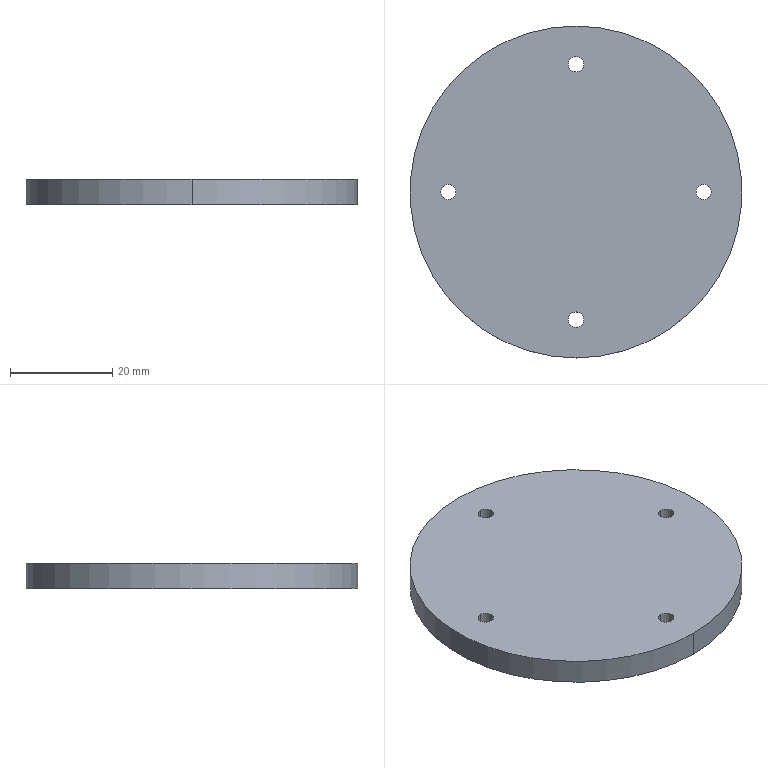Component | SolidWorks | Gimbal-1_GimbalMiddle-1 | 1 solid | 12 faces | box 65 x 65 x 5 mm | volume 16450 mm3 | cylinder 10 | plane 2 | commonest cylinder face diameters 3 x8 65 x2
build123d program:
from build123d import *

# Parameters (mm, degrees)
SKETCH1_R           = 32.5
BOSS_EXTRUDE1_DEPTH = 5
SKETCH2_R           = 1.5
CUT_EXTRUDE3_DEPTH  = 10


with BuildPart() as part:
    # Sketch1 → Boss-Extrude1 (new body)
    with BuildSketch(Plane.XY):
        Circle(SKETCH1_R)
    extrude(amount=BOSS_EXTRUDE1_DEPTH)

    # Sketch2 → Cut-Extrude3 (cut)
    with BuildSketch(Plane.XY.offset(5)):
        with Locations((0, 25)):
            Circle(SKETCH2_R)
        with Locations((25, 0)):
            Circle(SKETCH2_R)
        with Locations((0, -25)):
            Circle(SKETCH2_R)
        with Locations((-25, 0)):
            Circle(SKETCH2_R)
    extrude(amount=-CUT_EXTRUDE3_DEPTH, mode=Mode.SUBTRACT)


solid = part.part

# Placed as in the assembly
solid = solid.moved(Location((0, 96.5, -37), (0, 0, 0)))
STEP:
#1=COLOUR_RGB('',0.7922,0.8196,0.9333);
#2=FILL_AREA_STYLE_COLOUR('',#1);
#3=FILL_AREA_STYLE('',(#2));
#4=SURFACE_STYLE_FILL_AREA(#3);
#5=SURFACE_SIDE_STYLE('',(#4));
#6=SURFACE_STYLE_USAGE(.BOTH.,#5);
#7=PRESENTATION_STYLE_ASSIGNMENT((#6));
#8=CARTESIAN_POINT('',(-0.9843,3.858,-1.26));
#9=VERTEX_POINT('',#8);
#10=CARTESIAN_POINT('',(-0.9843,3.74,-1.26));
#11=VERTEX_POINT('',#10);
#12=CARTESIAN_POINT('',(-0.9843,3.799,-1.26));
#13=DIRECTION('',(0.,0.,-1.));
#14=DIRECTION('',(0.,-1.,0.));
#15=AXIS2_PLACEMENT_3D('',#12,#13,#14);
#16=CIRCLE('',#15,0.05906);
#17=EDGE_CURVE('',#9,#11,#16,.T.);
#18=ORIENTED_EDGE('',*,*,#17,.F.);
#19=CARTESIAN_POINT('',(-0.9843,3.858,-1.457));
#20=VERTEX_POINT('',#19);
#21=CARTESIAN_POINT('',(-0.9843,3.858,-1.063));
#22=DIRECTION('',(0.,0.,-1.));
#23=VECTOR('',#22,39.37);
#24=LINE('',#21,#23);
#25=EDGE_CURVE('',#9,#20,#24,.T.);
#26=ORIENTED_EDGE('',*,*,#25,.T.);
#27=CARTESIAN_POINT('',(-0.9843,3.74,-1.457));
#28=VERTEX_POINT('',#27);
#29=CARTESIAN_POINT('',(-0.9843,3.799,-1.457));
#30=DIRECTION('',(0.,0.,-1.));
#31=DIRECTION('',(0.,-1.,0.));
#32=AXIS2_PLACEMENT_3D('',#29,#30,#31);
#33=CIRCLE('',#32,0.05906);
#34=EDGE_CURVE('',#20,#28,#33,.T.);
#35=ORIENTED_EDGE('',*,*,#34,.T.);
#36=CARTESIAN_POINT('',(-0.9843,3.74,-1.063));
#37=DIRECTION('',(0.,0.,-1.));
#38=VECTOR('',#37,39.37);
#39=LINE('',#36,#38);
#40=EDGE_CURVE('',#11,#28,#39,.T.);
#41=ORIENTED_EDGE('',*,*,#40,.F.);
#42=EDGE_LOOP('',(#18,#26,#35,#41));
#43=FACE_OUTER_BOUND('',#42,.T.);
#44=CARTESIAN_POINT('',(-0.9843,3.799,-1.063));
#45=DIRECTION('',(0.,0.,-1.));
#46=DIRECTION('',(0.,-1.,0.));
#47=AXIS2_PLACEMENT_3D('',#44,#45,#46);
#48=CYLINDRICAL_SURFACE('',#47,0.05906);
#49=ADVANCED_FACE('',(#43),#48,.F.);
#50=CARTESIAN_POINT('',(0.,2.874,-1.26));
#51=VERTEX_POINT('',#50);
#52=CARTESIAN_POINT('',(0.,2.756,-1.26));
#53=VERTEX_POINT('',#52);
#54=CARTESIAN_POINT('',(0.,2.815,-1.26));
#55=DIRECTION('',(0.,0.,-1.));
#56=DIRECTION('',(0.,-1.,0.));
#57=AXIS2_PLACEMENT_3D('',#54,#55,#56);
#58=CIRCLE('',#57,0.05906);
#59=EDGE_CURVE('',#51,#53,#58,.T.);
#60=ORIENTED_EDGE('',*,*,#59,.F.);
#61=CARTESIAN_POINT('',(0.,2.874,-1.457));
#62=VERTEX_POINT('',#61);
#63=CARTESIAN_POINT('',(0.,2.874,-1.063));
#64=DIRECTION('',(0.,0.,-1.));
#65=VECTOR('',#64,39.37);
#66=LINE('',#63,#65);
#67=EDGE_CURVE('',#51,#62,#66,.T.);
#68=ORIENTED_EDGE('',*,*,#67,.T.);
#69=CARTESIAN_POINT('',(0.,2.756,-1.457));
#70=VERTEX_POINT('',#69);
#71=CARTESIAN_POINT('',(0.,2.815,-1.457));
#72=DIRECTION('',(0.,0.,-1.));
#73=DIRECTION('',(0.,-1.,0.));
#74=AXIS2_PLACEMENT_3D('',#71,#72,#73);
#75=CIRCLE('',#74,0.05906);
#76=EDGE_CURVE('',#62,#70,#75,.T.);
#77=ORIENTED_EDGE('',*,*,#76,.T.);
#78=CARTESIAN_POINT('',(0.,2.756,-1.063));
#79=DIRECTION('',(0.,0.,-1.));
#80=VECTOR('',#79,39.37);
#81=LINE('',#78,#80);
#82=EDGE_CURVE('',#53,#70,#81,.T.);
#83=ORIENTED_EDGE('',*,*,#82,.F.);
#84=EDGE_LOOP('',(#60,#68,#77,#83));
#85=FACE_OUTER_BOUND('',#84,.T.);
#86=CARTESIAN_POINT('',(0.,2.815,-1.063));
#87=DIRECTION('',(0.,0.,-1.));
#88=DIRECTION('',(0.,-1.,0.));
#89=AXIS2_PLACEMENT_3D('',#86,#87,#88);
#90=CYLINDRICAL_SURFACE('',#89,0.05906);
#91=ADVANCED_FACE('',(#85),#90,.F.);
#92=CARTESIAN_POINT('',(0.9843,3.858,-1.26));
#93=VERTEX_POINT('',#92);
#94=CARTESIAN_POINT('',(0.9843,3.74,-1.26));
#95=VERTEX_POINT('',#94);
#96=CARTESIAN_POINT('',(0.9843,3.799,-1.26));
#97=DIRECTION('',(0.,0.,-1.));
#98=DIRECTION('',(0.,-1.,0.));
#99=AXIS2_PLACEMENT_3D('',#96,#97,#98);
#100=CIRCLE('',#99,0.05906);
#101=EDGE_CURVE('',#93,#95,#100,.T.);
#102=ORIENTED_EDGE('',*,*,#101,.F.);
#103=CARTESIAN_POINT('',(0.9843,3.858,-1.457));
#104=VERTEX_POINT('',#103);
#105=CARTESIAN_POINT('',(0.9843,3.858,-1.063));
#106=DIRECTION('',(0.,0.,-1.));
#107=VECTOR('',#106,39.37);
#108=LINE('',#105,#107);
#109=EDGE_CURVE('',#93,#104,#108,.T.);
#110=ORIENTED_EDGE('',*,*,#109,.T.);
#111=CARTESIAN_POINT('',(0.9843,3.74,-1.457));
#112=VERTEX_POINT('',#111);
#113=CARTESIAN_POINT('',(0.9843,3.799,-1.457));
#114=DIRECTION('',(0.,0.,-1.));
#115=DIRECTION('',(0.,-1.,0.));
#116=AXIS2_PLACEMENT_3D('',#113,#114,#115);
#117=CIRCLE('',#116,0.05906);
#118=EDGE_CURVE('',#104,#112,#117,.T.);
#119=ORIENTED_EDGE('',*,*,#118,.T.);
#120=CARTESIAN_POINT('',(0.9843,3.74,-1.063));
#121=DIRECTION('',(0.,0.,-1.));
#122=VECTOR('',#121,39.37);
#123=LINE('',#120,#122);
#124=EDGE_CURVE('',#95,#112,#123,.T.);
#125=ORIENTED_EDGE('',*,*,#124,.F.);
#126=EDGE_LOOP('',(#102,#110,#119,#125));
#127=FACE_OUTER_BOUND('',#126,.T.);
#128=CARTESIAN_POINT('',(0.9843,3.799,-1.063));
#129=DIRECTION('',(0.,0.,-1.));
#130=DIRECTION('',(0.,-1.,0.));
#131=AXIS2_PLACEMENT_3D('',#128,#129,#130);
#132=CYLINDRICAL_SURFACE('',#131,0.05906);
#133=ADVANCED_FACE('',(#127),#132,.F.);
#134=CARTESIAN_POINT('',(-0.,4.843,-1.26));
#135=VERTEX_POINT('',#134);
#136=CARTESIAN_POINT('',(-0.,4.724,-1.26));
#137=VERTEX_POINT('',#136);
#138=CARTESIAN_POINT('',(-0.,4.783,-1.26));
#139=DIRECTION('',(0.,0.,-1.));
#140=DIRECTION('',(0.,-1.,0.));
#141=AXIS2_PLACEMENT_3D('',#138,#139,#140);
#142=CIRCLE('',#141,0.05906);
#143=EDGE_CURVE('',#135,#137,#142,.T.);
#144=ORIENTED_EDGE('',*,*,#143,.F.);
#145=CARTESIAN_POINT('',(-0.,4.843,-1.457));
#146=VERTEX_POINT('',#145);
#147=CARTESIAN_POINT('',(-0.,4.843,-1.063));
#148=DIRECTION('',(0.,0.,-1.));
#149=VECTOR('',#148,39.37);
#150=LINE('',#147,#149);
#151=EDGE_CURVE('',#135,#146,#150,.T.);
#152=ORIENTED_EDGE('',*,*,#151,.T.);
#153=CARTESIAN_POINT('',(-0.,4.724,-1.457));
#154=VERTEX_POINT('',#153);
#155=CARTESIAN_POINT('',(-0.,4.783,-1.457));
#156=DIRECTION('',(0.,0.,-1.));
#157=DIRECTION('',(0.,-1.,0.));
#158=AXIS2_PLACEMENT_3D('',#155,#156,#157);
#159=CIRCLE('',#158,0.05906);
#160=EDGE_CURVE('',#146,#154,#159,.T.);
#161=ORIENTED_EDGE('',*,*,#160,.T.);
#162=CARTESIAN_POINT('',(-0.,4.724,-1.063));
#163=DIRECTION('',(0.,0.,-1.));
#164=VECTOR('',#163,39.37);
#165=LINE('',#162,#164);
#166=EDGE_CURVE('',#137,#154,#165,.T.);
#167=ORIENTED_EDGE('',*,*,#166,.F.);
#168=EDGE_LOOP('',(#144,#152,#161,#167));
#169=FACE_OUTER_BOUND('',#168,.T.);
#170=CARTESIAN_POINT('',(-0.,4.783,-1.063));
#171=DIRECTION('',(0.,0.,-1.));
#172=DIRECTION('',(0.,-1.,0.));
#173=AXIS2_PLACEMENT_3D('',#170,#171,#172);
#174=CYLINDRICAL_SURFACE('',#173,0.05906);
#175=ADVANCED_FACE('',(#169),#174,.F.);
#176=CARTESIAN_POINT('',(0.,2.52,-1.457));
#177=VERTEX_POINT('',#176);
#178=CARTESIAN_POINT('',(-0.,5.079,-1.457));
#179=VERTEX_POINT('',#178);
#180=CARTESIAN_POINT('',(0.,3.799,-1.457));
#181=DIRECTION('',(0.,0.,-1.));
#182=DIRECTION('',(0.,-1.,0.));
#183=AXIS2_PLACEMENT_3D('',#180,#181,#182);
#184=CIRCLE('',#183,1.28);
#185=EDGE_CURVE('',#177,#179,#184,.T.);
#186=ORIENTED_EDGE('',*,*,#185,.F.);
#187=CARTESIAN_POINT('',(0.,2.52,-1.26));
#188=VERTEX_POINT('',#187);
#189=CARTESIAN_POINT('',(0.,2.52,-1.457));
#190=DIRECTION('',(0.,0.,1.));
#191=VECTOR('',#190,39.37);
#192=LINE('',#189,#191);
#193=EDGE_CURVE('',#177,#188,#192,.T.);
#194=ORIENTED_EDGE('',*,*,#193,.T.);
#195=CARTESIAN_POINT('',(-0.,5.079,-1.26));
#196=VERTEX_POINT('',#195);
#197=CARTESIAN_POINT('',(0.,3.799,-1.26));
#198=DIRECTION('',(0.,0.,-1.));
#199=DIRECTION('',(0.,-1.,0.));
#200=AXIS2_PLACEMENT_3D('',#197,#198,#199);
#201=CIRCLE('',#200,1.28);
#202=EDGE_CURVE('',#188,#196,#201,.T.);
#203=ORIENTED_EDGE('',*,*,#202,.T.);
#204=CARTESIAN_POINT('',(-0.,5.079,-1.457));
#205=DIRECTION('',(0.,0.,1.));
#206=VECTOR('',#205,39.37);
#207=LINE('',#204,#206);
#208=EDGE_CURVE('',#179,#196,#207,.T.);
#209=ORIENTED_EDGE('',*,*,#208,.F.);
#210=EDGE_LOOP('',(#186,#194,#203,#209));
#211=FACE_OUTER_BOUND('',#210,.T.);
#212=CARTESIAN_POINT('',(0.,3.799,-1.457));
#213=DIRECTION('',(0.,0.,1.));
#214=DIRECTION('',(-0.,1.,0.));
#215=AXIS2_PLACEMENT_3D('',#212,#213,#214);
#216=CYLINDRICAL_SURFACE('',#215,1.28);
#217=ADVANCED_FACE('',(#211),#216,.T.);
#218=ORIENTED_EDGE('',*,*,#193,.F.);
#219=CARTESIAN_POINT('',(0.,3.799,-1.457));
#220=DIRECTION('',(0.,0.,-1.));
#221=DIRECTION('',(0.,-1.,0.));
#222=AXIS2_PLACEMENT_3D('',#219,#220,#221);
#223=CIRCLE('',#222,1.28);
#224=EDGE_CURVE('',#179,#177,#223,.T.);
#225=ORIENTED_EDGE('',*,*,#224,.F.);
#226=ORIENTED_EDGE('',*,*,#208,.T.);
#227=CARTESIAN_POINT('',(0.,3.799,-1.26));
#228=DIRECTION('',(0.,0.,-1.));
#229=DIRECTION('',(0.,-1.,0.));
#230=AXIS2_PLACEMENT_3D('',#227,#228,#229);
#231=CIRCLE('',#230,1.28);
#232=EDGE_CURVE('',#196,#188,#231,.T.);
#233=ORIENTED_EDGE('',*,*,#232,.T.);
#234=EDGE_LOOP('',(#218,#225,#226,#233));
#235=FACE_OUTER_BOUND('',#234,.T.);
#236=CARTESIAN_POINT('',(0.,3.799,-1.457));
#237=DIRECTION('',(0.,0.,1.));
#238=DIRECTION('',(-0.,1.,0.));
#239=AXIS2_PLACEMENT_3D('',#236,#237,#238);
#240=CYLINDRICAL_SURFACE('',#239,1.28);
#241=ADVANCED_FACE('',(#235),#240,.T.);
#242=CARTESIAN_POINT('',(-0.9843,3.799,-1.457));
#243=DIRECTION('',(0.,0.,-1.));
#244=DIRECTION('',(0.,-1.,0.));
#245=AXIS2_PLACEMENT_3D('',#242,#243,#244);
#246=CIRCLE('',#245,0.05906);
#247=EDGE_CURVE('',#28,#20,#246,.T.);
#248=ORIENTED_EDGE('',*,*,#247,.F.);
#249=ORIENTED_EDGE('',*,*,#34,.F.);
#250=EDGE_LOOP('',(#248,#249));
#251=FACE_BOUND('',#250,.T.);
#252=CARTESIAN_POINT('',(0.,2.815,-1.457));
#253=DIRECTION('',(0.,0.,-1.));
#254=DIRECTION('',(0.,-1.,0.));
#255=AXIS2_PLACEMENT_3D('',#252,#253,#254);
#256=CIRCLE('',#255,0.05906);
#257=EDGE_CURVE('',#70,#62,#256,.T.);
#258=ORIENTED_EDGE('',*,*,#257,.F.);
#259=ORIENTED_EDGE('',*,*,#76,.F.);
#260=EDGE_LOOP('',(#258,#259));
#261=FACE_BOUND('',#260,.T.);
#262=CARTESIAN_POINT('',(0.9843,3.799,-1.457));
#263=DIRECTION('',(0.,0.,-1.));
#264=DIRECTION('',(0.,-1.,0.));
#265=AXIS2_PLACEMENT_3D('',#262,#263,#264);
#266=CIRCLE('',#265,0.05906);
#267=EDGE_CURVE('',#112,#104,#266,.T.);
#268=ORIENTED_EDGE('',*,*,#267,.F.);
#269=ORIENTED_EDGE('',*,*,#118,.F.);
#270=EDGE_LOOP('',(#268,#269));
#271=FACE_BOUND('',#270,.T.);
#272=CARTESIAN_POINT('',(-0.,4.783,-1.457));
#273=DIRECTION('',(0.,0.,-1.));
#274=DIRECTION('',(0.,-1.,0.));
#275=AXIS2_PLACEMENT_3D('',#272,#273,#274);
#276=CIRCLE('',#275,0.05906);
#277=EDGE_CURVE('',#154,#146,#276,.T.);
#278=ORIENTED_EDGE('',*,*,#277,.F.);
#279=ORIENTED_EDGE('',*,*,#160,.F.);
#280=EDGE_LOOP('',(#278,#279));
#281=FACE_BOUND('',#280,.T.);
#282=ORIENTED_EDGE('',*,*,#224,.T.);
#283=ORIENTED_EDGE('',*,*,#185,.T.);
#284=EDGE_LOOP('',(#282,#283));
#285=FACE_OUTER_BOUND('',#284,.T.);
#286=CARTESIAN_POINT('',(0.,3.799,-1.457));
#287=DIRECTION('',(0.,0.,-1.));
#288=DIRECTION('',(0.,-1.,0.));
#289=AXIS2_PLACEMENT_3D('',#286,#287,#288);
#290=PLANE('',#289);
#291=ADVANCED_FACE('',(#251,#261,#271,#281,#285),#290,.T.);
#292=CARTESIAN_POINT('',(-0.9843,3.799,-1.26));
#293=DIRECTION('',(0.,0.,-1.));
#294=DIRECTION('',(0.,-1.,0.));
#295=AXIS2_PLACEMENT_3D('',#292,#293,#294);
#296=CIRCLE('',#295,0.05906);
#297=EDGE_CURVE('',#11,#9,#296,.T.);
#298=ORIENTED_EDGE('',*,*,#297,.T.);
#299=ORIENTED_EDGE('',*,*,#17,.T.);
#300=EDGE_LOOP('',(#298,#299));
#301=FACE_BOUND('',#300,.T.);
#302=CARTESIAN_POINT('',(0.,2.815,-1.26));
#303=DIRECTION('',(0.,0.,-1.));
#304=DIRECTION('',(0.,-1.,0.));
#305=AXIS2_PLACEMENT_3D('',#302,#303,#304);
#306=CIRCLE('',#305,0.05906);
#307=EDGE_CURVE('',#53,#51,#306,.T.);
#308=ORIENTED_EDGE('',*,*,#307,.T.);
#309=ORIENTED_EDGE('',*,*,#59,.T.);
#310=EDGE_LOOP('',(#308,#309));
#311=FACE_BOUND('',#310,.T.);
#312=CARTESIAN_POINT('',(0.9843,3.799,-1.26));
#313=DIRECTION('',(0.,0.,-1.));
#314=DIRECTION('',(0.,-1.,0.));
#315=AXIS2_PLACEMENT_3D('',#312,#313,#314);
#316=CIRCLE('',#315,0.05906);
#317=EDGE_CURVE('',#95,#93,#316,.T.);
#318=ORIENTED_EDGE('',*,*,#317,.T.);
#319=ORIENTED_EDGE('',*,*,#101,.T.);
#320=EDGE_LOOP('',(#318,#319));
#321=FACE_BOUND('',#320,.T.);
#322=CARTESIAN_POINT('',(-0.,4.783,-1.26));
#323=DIRECTION('',(0.,0.,-1.));
#324=DIRECTION('',(0.,-1.,0.));
#325=AXIS2_PLACEMENT_3D('',#322,#323,#324);
#326=CIRCLE('',#325,0.05906);
#327=EDGE_CURVE('',#137,#135,#326,.T.);
#328=ORIENTED_EDGE('',*,*,#327,.T.);
#329=ORIENTED_EDGE('',*,*,#143,.T.);
#330=EDGE_LOOP('',(#328,#329));
#331=FACE_BOUND('',#330,.T.);
#332=ORIENTED_EDGE('',*,*,#232,.F.);
#333=ORIENTED_EDGE('',*,*,#202,.F.);
#334=EDGE_LOOP('',(#332,#333));
#335=FACE_OUTER_BOUND('',#334,.T.);
#336=CARTESIAN_POINT('',(0.,3.799,-1.26));
#337=DIRECTION('',(0.,0.,-1.));
#338=DIRECTION('',(0.,-1.,0.));
#339=AXIS2_PLACEMENT_3D('',#336,#337,#338);
#340=PLANE('',#339);
#341=ADVANCED_FACE('',(#301,#311,#321,#331,#335),#340,.F.);
#342=ORIENTED_EDGE('',*,*,#151,.F.);
#343=ORIENTED_EDGE('',*,*,#327,.F.);
#344=ORIENTED_EDGE('',*,*,#166,.T.);
#345=ORIENTED_EDGE('',*,*,#277,.T.);
#346=EDGE_LOOP('',(#342,#343,#344,#345));
#347=FACE_OUTER_BOUND('',#346,.T.);
#348=CARTESIAN_POINT('',(-0.,4.783,-1.063));
#349=DIRECTION('',(0.,0.,-1.));
#350=DIRECTION('',(0.,-1.,0.));
#351=AXIS2_PLACEMENT_3D('',#348,#349,#350);
#352=CYLINDRICAL_SURFACE('',#351,0.05906);
#353=ADVANCED_FACE('',(#347),#352,.F.);
#354=ORIENTED_EDGE('',*,*,#109,.F.);
#355=ORIENTED_EDGE('',*,*,#317,.F.);
#356=ORIENTED_EDGE('',*,*,#124,.T.);
#357=ORIENTED_EDGE('',*,*,#267,.T.);
#358=EDGE_LOOP('',(#354,#355,#356,#357));
#359=FACE_OUTER_BOUND('',#358,.T.);
#360=CARTESIAN_POINT('',(0.9843,3.799,-1.063));
#361=DIRECTION('',(0.,0.,-1.));
#362=DIRECTION('',(0.,-1.,0.));
#363=AXIS2_PLACEMENT_3D('',#360,#361,#362);
#364=CYLINDRICAL_SURFACE('',#363,0.05906);
#365=ADVANCED_FACE('',(#359),#364,.F.);
#366=ORIENTED_EDGE('',*,*,#67,.F.);
#367=ORIENTED_EDGE('',*,*,#307,.F.);
#368=ORIENTED_EDGE('',*,*,#82,.T.);
#369=ORIENTED_EDGE('',*,*,#257,.T.);
#370=EDGE_LOOP('',(#366,#367,#368,#369));
#371=FACE_OUTER_BOUND('',#370,.T.);
#372=CARTESIAN_POINT('',(0.,2.815,-1.063));
#373=DIRECTION('',(0.,0.,-1.));
#374=DIRECTION('',(0.,-1.,0.));
#375=AXIS2_PLACEMENT_3D('',#372,#373,#374);
#376=CYLINDRICAL_SURFACE('',#375,0.05906);
#377=ADVANCED_FACE('',(#371),#376,.F.);
#378=ORIENTED_EDGE('',*,*,#25,.F.);
#379=ORIENTED_EDGE('',*,*,#297,.F.);
#380=ORIENTED_EDGE('',*,*,#40,.T.);
#381=ORIENTED_EDGE('',*,*,#247,.T.);
#382=EDGE_LOOP('',(#378,#379,#380,#381));
#383=FACE_OUTER_BOUND('',#382,.T.);
#384=CARTESIAN_POINT('',(-0.9843,3.799,-1.063));
#385=DIRECTION('',(0.,0.,-1.));
#386=DIRECTION('',(0.,-1.,0.));
#387=AXIS2_PLACEMENT_3D('',#384,#385,#386);
#388=CYLINDRICAL_SURFACE('',#387,0.05906);
#389=ADVANCED_FACE('',(#383),#388,.F.);
#390=CLOSED_SHELL('',(#49,#91,#133,#175,#217,#241,#291,#341,#353,#365,#377,#389));
#391=MANIFOLD_SOLID_BREP('',#390);
#392=STYLED_ITEM('',(#7),#391);
#393=(LENGTH_UNIT()NAMED_UNIT(*)SI_UNIT($,.METRE.));
#394=LENGTH_MEASURE_WITH_UNIT(LENGTH_MEASURE(0.0254),#393);
#395=DIMENSIONAL_EXPONENTS(1.,0.,0.,0.,0.,0.,0.);
#396=(CONVERSION_BASED_UNIT('',#394)LENGTH_UNIT()NAMED_UNIT(#395));
#397=UNCERTAINTY_MEASURE_WITH_UNIT(LENGTH_MEASURE(0.00001),#396,'','');
#398=(NAMED_UNIT(*)PLANE_ANGLE_UNIT()SI_UNIT($,.RADIAN.));
#399=(NAMED_UNIT(*)SI_UNIT($,.STERADIAN.)SOLID_ANGLE_UNIT());
#400=(GEOMETRIC_REPRESENTATION_CONTEXT(3)GLOBAL_UNCERTAINTY_ASSIGNED_CONTEXT((#397))GLOBAL_UNIT_ASSIGNED_CONTEXT((#396,#398,#399))REPRESENTATION_CONTEXT('',''));
#401=MECHANICAL_DESIGN_GEOMETRIC_PRESENTATION_REPRESENTATION('',(#392),#400);
#402=CARTESIAN_POINT('',(0.,0.,0.));
#403=DIRECTION('',(0.,0.,1.));
#404=DIRECTION('',(1.,0.,0.));
#405=AXIS2_PLACEMENT_3D('',#402,#403,#404);
#406=(LENGTH_UNIT()NAMED_UNIT(*)SI_UNIT($,.METRE.));
#407=LENGTH_MEASURE_WITH_UNIT(LENGTH_MEASURE(0.0254),#406);
#408=DIMENSIONAL_EXPONENTS(1.,0.,0.,0.,0.,0.,0.);
#409=(CONVERSION_BASED_UNIT('',#407)LENGTH_UNIT()NAMED_UNIT(#408));
#410=UNCERTAINTY_MEASURE_WITH_UNIT(LENGTH_MEASURE(0.00001),#409,'','');
#411=(NAMED_UNIT(*)PLANE_ANGLE_UNIT()SI_UNIT($,.RADIAN.));
#412=(NAMED_UNIT(*)SI_UNIT($,.STERADIAN.)SOLID_ANGLE_UNIT());
#413=(GEOMETRIC_REPRESENTATION_CONTEXT(3)GLOBAL_UNCERTAINTY_ASSIGNED_CONTEXT((#410))GLOBAL_UNIT_ASSIGNED_CONTEXT((#409,#411,#412))REPRESENTATION_CONTEXT('',''));
#414=ADVANCED_BREP_SHAPE_REPRESENTATION('',(#391,#405),#413);
#415=PRESENTATION_LAYER_ASSIGNMENT('','',(#392));